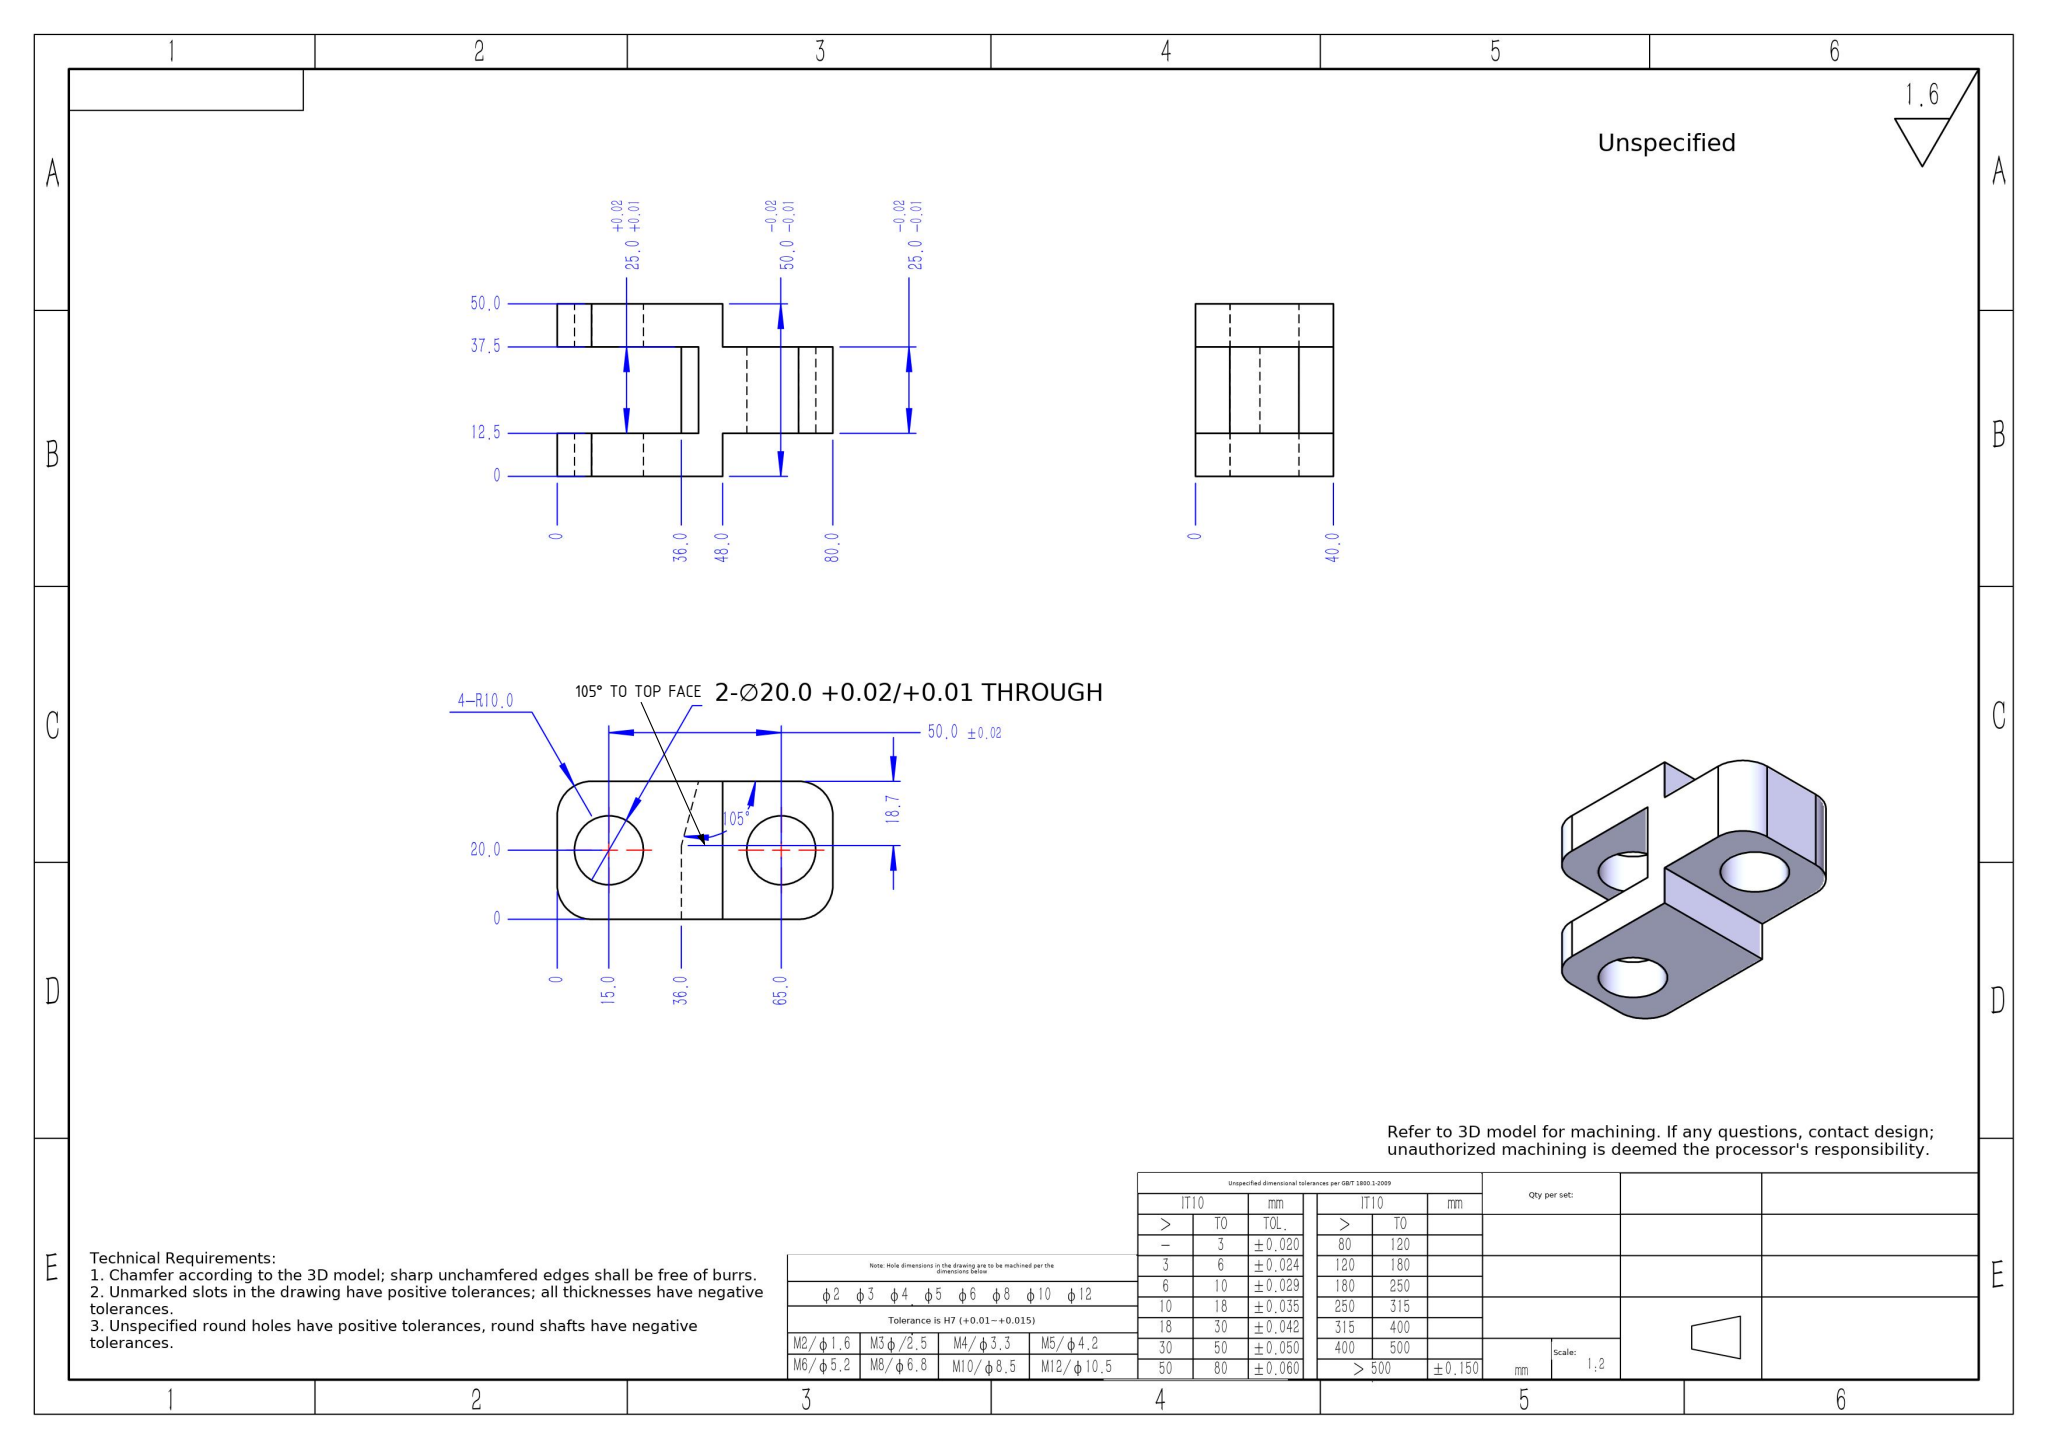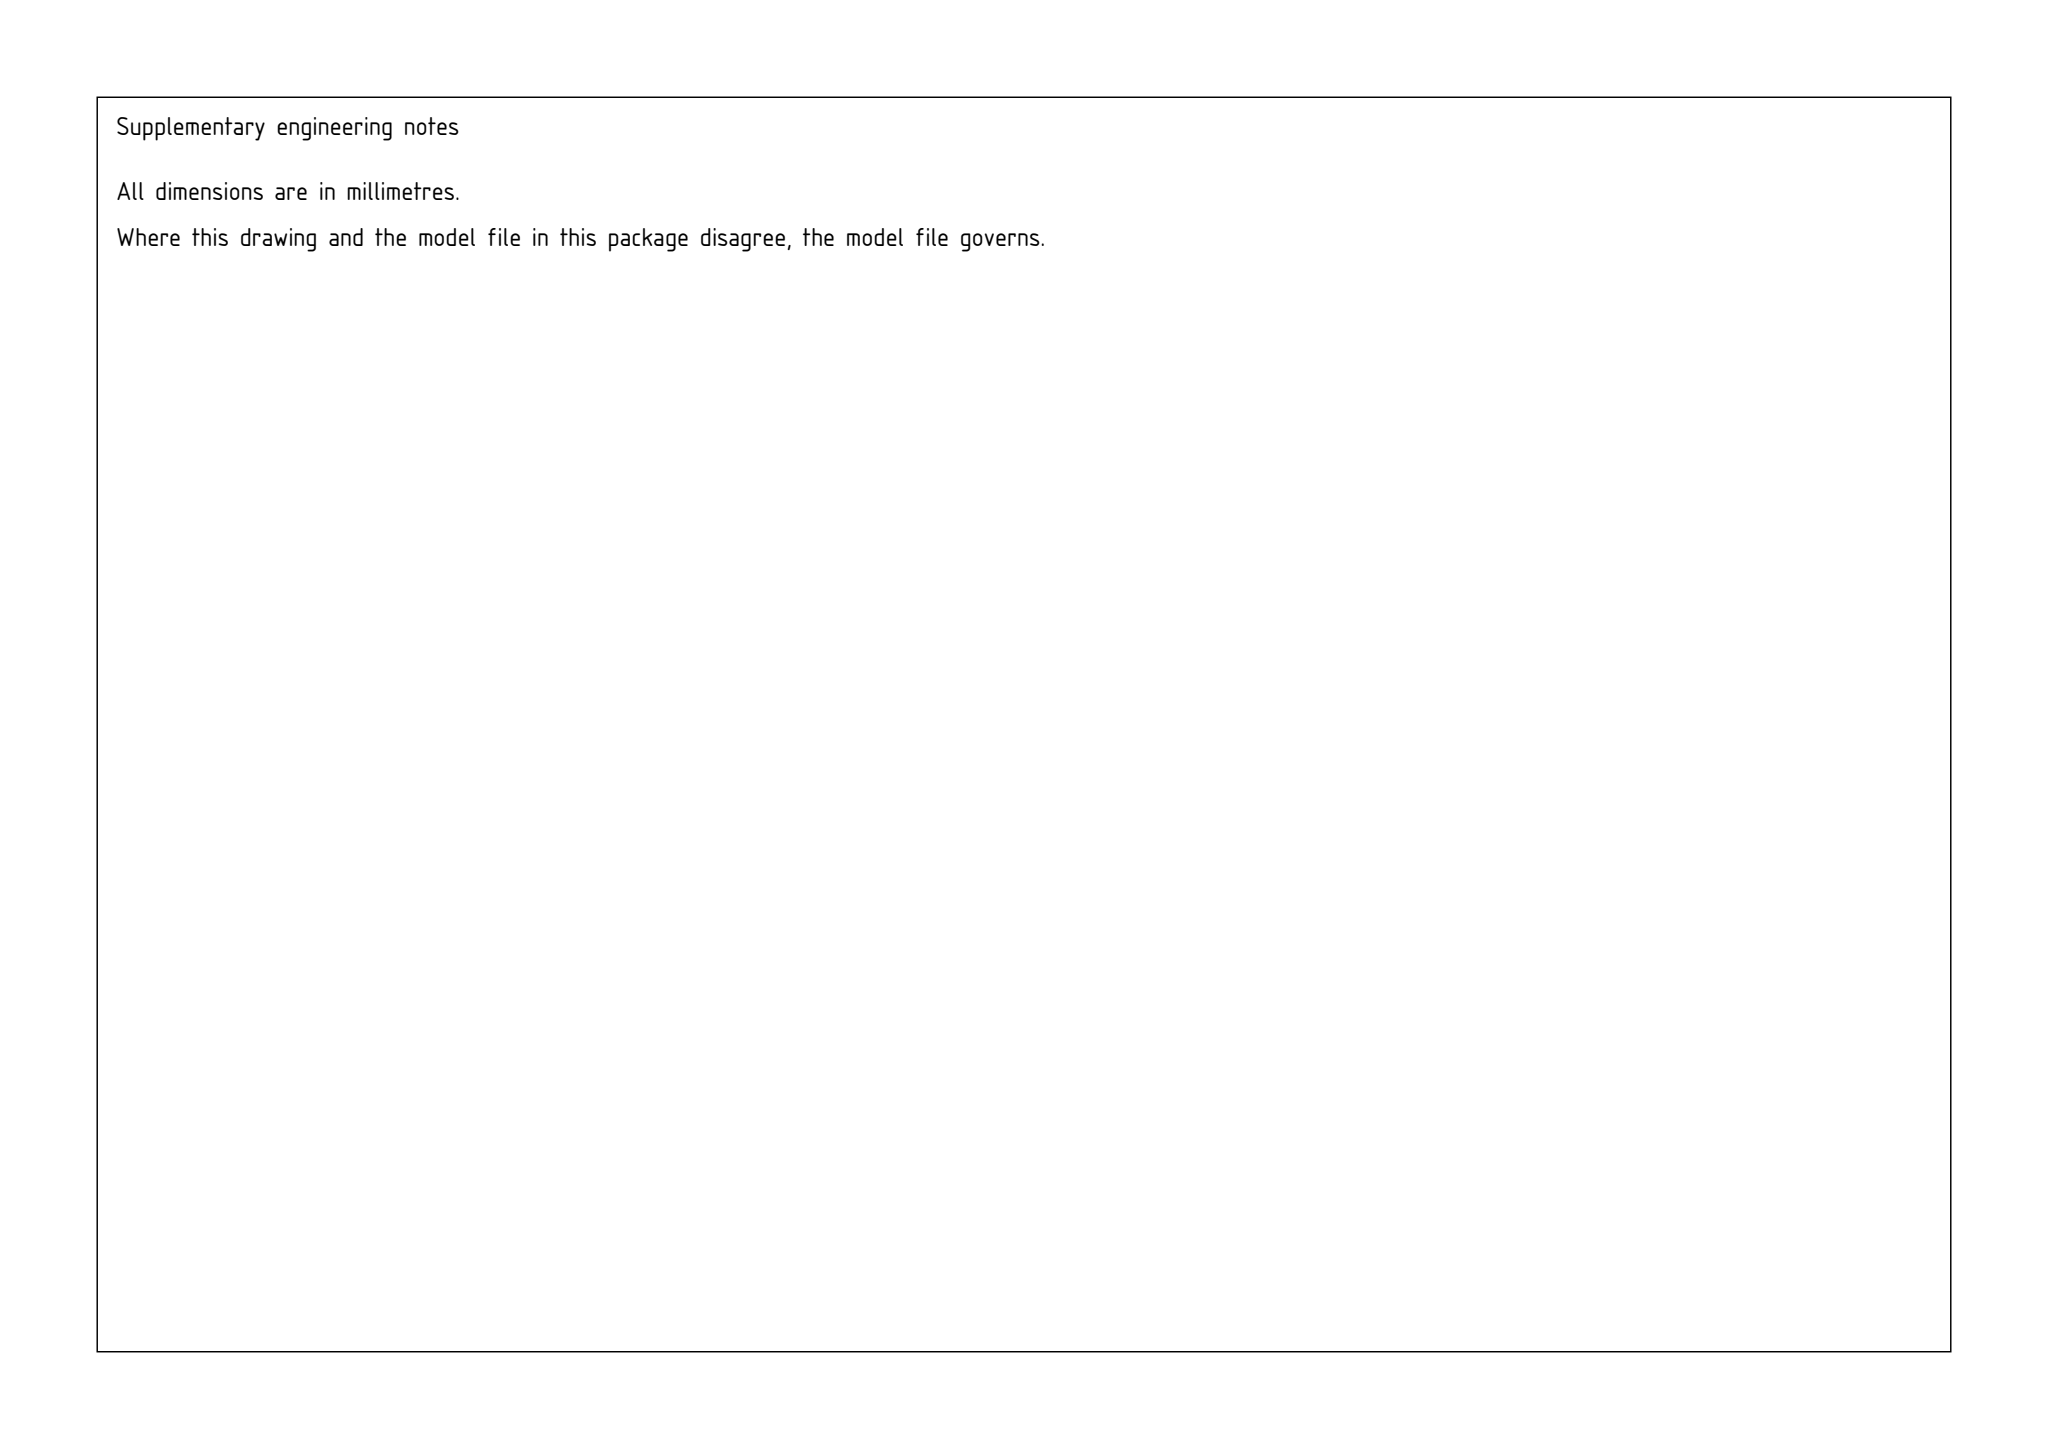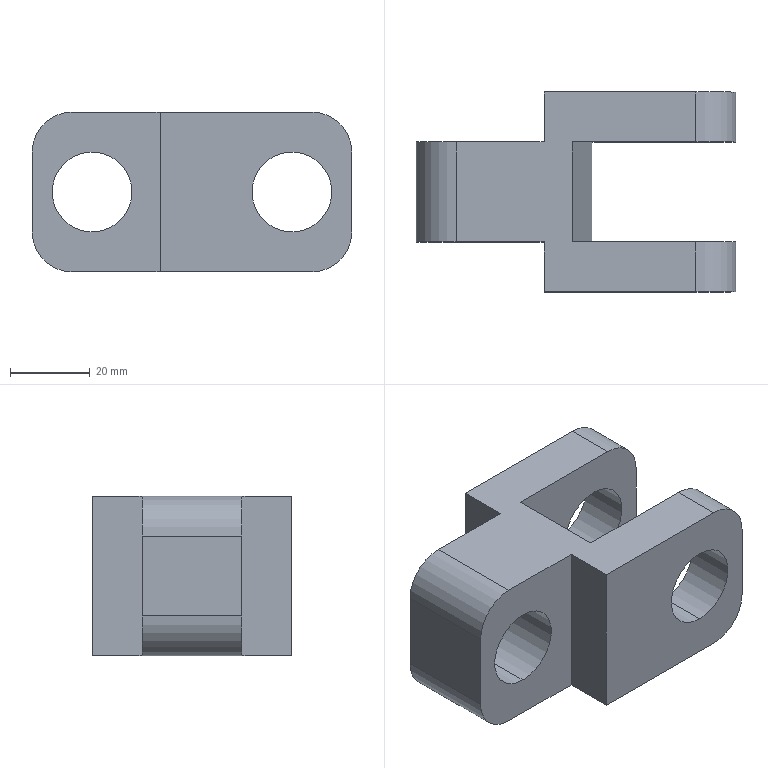Part | SolidWorks | mm | 1 solid | 27 faces | box 80 x 50 x 40 mm | volume 72980 mm3 | plane 15 | cylinder 12 | commonest cylinder face diameters 20 x12
Drawing notes:
ANGLED FACE 105° TO TOP FACE; RISE 18.7 OVER 5.0 RUN | from the solid: inclined plane angle_to_xyz [15,90,75], bbox_from [39,12.5,21.3], size [5,25,18.7]; 180-atan(18.7/5)=105° from top face z=40
build123d program:
from build123d import *

# Parameters (mm, degrees)
SKETCH1_W           = 80
SKETCH1_H           = 50
BOSS_EXTRUDE1_DEPTH = 20
SKETCH2_R           = 10
CUT_EXTRUDE1_DEPTH  = 205
SKETCH3_W           = 32
SKETCH3_H           = 40
CUT_EXTRUDE2_DEPTH  = 12.5
SKETCH4_W           = 36
SKETCH4_H           = 25
CUT_EXTRUDE3_DEPTH  = 256
FILLET1_R           = 10
CHAMFER1_SIZE       = 5
CHAMFER1_SIZE2      = 18.66


with BuildPart() as part:
    # Sketch1 → Boss-Extrude1 (new, symmetric)
    with BuildSketch(Plane.XY):
        Rectangle(SKETCH1_W, SKETCH1_H)
    extrude(amount=BOSS_EXTRUDE1_DEPTH, both=True)

    # Sketch2 → Cut-Extrude1 (cut)
    with BuildSketch(Plane.XZ.offset(25)):
        with Locations(Location((25, 0, 0), (0, 0, 270))):
            Circle(SKETCH2_R)
    cut_extrude1 = extrude(amount=-CUT_EXTRUDE1_DEPTH, mode=Mode.SUBTRACT)

    # Mirror1: Cut-Extrude1 across plane
    add(cut_extrude1.mirror(Plane(origin=(0, 0, 0), x_dir=(0, 0, 1), z_dir=(1, 0, 0))), mode=Mode.SUBTRACT)

    # Sketch3 → Cut-Extrude2 (cut)
    with BuildSketch(Plane.XZ.offset(25)):
        with Locations((-24, 0)):
            Rectangle(SKETCH3_W, SKETCH3_H)
    cut_extrude2 = extrude(amount=-CUT_EXTRUDE2_DEPTH, mode=Mode.SUBTRACT)

    # Mirror2: Cut-Extrude2 across plane
    add(cut_extrude2.mirror(Plane.ZX), mode=Mode.SUBTRACT)

    # Sketch4 → Cut-Extrude3 (cut)
    with BuildSketch(Plane(origin=(0, 0, -20), x_dir=(-1, 0, 0), z_dir=(0, 0, -1))):
        with Locations((-22, 0)):
            Rectangle(SKETCH4_W, SKETCH4_H)
    extrude(amount=-CUT_EXTRUDE3_DEPTH, mode=Mode.SUBTRACT)

    # Fillet1
    fillet1_edges = [part.edges().sort_by_distance(p)[0] for p in [
        (40, -18.75, 20),
        (-40, 0, -20),
        (-40, 0, 20),
        (40, -18.75, -20),
        (40, 18.75, -20),
        (40, 18.75, 20),
    ]]
    fillet(fillet1_edges, radius=FILLET1_R)

    # Chamfer1
    chamfer1_edges = [part.edges().sort_by_distance(p)[0] for p in [
        (4, 0, 20),
    ]]
    chamfer1_side = [part.faces().sort_by_distance(p)[0] for p in [
        (-0.3333, 0, 20),
    ]]
    chamfer(chamfer1_edges, length=CHAMFER1_SIZE, length2=CHAMFER1_SIZE2, reference=chamfer1_side[0])


solid = part.part
STEP:
#1=CARTESIAN_POINT('',(25.,-12.5,-10.));
#2=VERTEX_POINT('',#1);
#3=CARTESIAN_POINT('',(25.,-12.5,10.));
#4=VERTEX_POINT('',#3);
#5=CARTESIAN_POINT('',(25.,-12.5,0.));
#6=DIRECTION('',(0.,1.,0.));
#7=DIRECTION('',(0.,0.,-1.));
#8=AXIS2_PLACEMENT_3D('',#5,#6,#7);
#9=CIRCLE('',#8,10.);
#10=EDGE_CURVE('',#2,#4,#9,.T.);
#11=ORIENTED_EDGE('',*,*,#10,.T.);
#12=CARTESIAN_POINT('',(25.,-25.,10.));
#13=VERTEX_POINT('',#12);
#14=CARTESIAN_POINT('',(25.,180.,10.));
#15=DIRECTION('',(0.,-1.,0.));
#16=VECTOR('',#15,1000.);
#17=LINE('',#14,#16);
#18=EDGE_CURVE('',#4,#13,#17,.T.);
#19=ORIENTED_EDGE('',*,*,#18,.T.);
#20=CARTESIAN_POINT('',(25.,-25.,-10.));
#21=VERTEX_POINT('',#20);
#22=CARTESIAN_POINT('',(25.,-25.,0.));
#23=DIRECTION('',(0.,-1.,0.));
#24=DIRECTION('',(0.,0.,-1.));
#25=AXIS2_PLACEMENT_3D('',#22,#23,#24);
#26=CIRCLE('',#25,10.);
#27=EDGE_CURVE('',#13,#21,#26,.T.);
#28=ORIENTED_EDGE('',*,*,#27,.T.);
#29=CARTESIAN_POINT('',(25.,180.,-10.));
#30=DIRECTION('',(0.,-1.,0.));
#31=VECTOR('',#30,1000.);
#32=LINE('',#29,#31);
#33=EDGE_CURVE('',#2,#21,#32,.T.);
#34=ORIENTED_EDGE('',*,*,#33,.F.);
#35=EDGE_LOOP('',(#11,#19,#28,#34));
#36=FACE_OUTER_BOUND('',#35,.T.);
#37=CARTESIAN_POINT('',(25.,180.,0.));
#38=DIRECTION('',(0.,-1.,0.));
#39=DIRECTION('',(0.,0.,-1.));
#40=AXIS2_PLACEMENT_3D('',#37,#38,#39);
#41=CYLINDRICAL_SURFACE('',#40,10.);
#42=ADVANCED_FACE('',(#36),#41,.F.);
#43=CARTESIAN_POINT('',(-25.,12.5,-10.));
#44=VERTEX_POINT('',#43);
#45=CARTESIAN_POINT('',(-25.,12.5,10.));
#46=VERTEX_POINT('',#45);
#47=CARTESIAN_POINT('',(-25.,12.5,0.));
#48=DIRECTION('',(0.,1.,0.));
#49=DIRECTION('',(0.,0.,1.));
#50=AXIS2_PLACEMENT_3D('',#47,#48,#49);
#51=CIRCLE('',#50,10.);
#52=EDGE_CURVE('',#44,#46,#51,.T.);
#53=ORIENTED_EDGE('',*,*,#52,.T.);
#54=CARTESIAN_POINT('',(-25.,-12.5,10.));
#55=VERTEX_POINT('',#54);
#56=CARTESIAN_POINT('',(-25.,180.,10.));
#57=DIRECTION('',(0.,-1.,0.));
#58=VECTOR('',#57,1000.);
#59=LINE('',#56,#58);
#60=EDGE_CURVE('',#46,#55,#59,.T.);
#61=ORIENTED_EDGE('',*,*,#60,.T.);
#62=CARTESIAN_POINT('',(-25.,-12.5,-10.));
#63=VERTEX_POINT('',#62);
#64=CARTESIAN_POINT('',(-25.,-12.5,0.));
#65=DIRECTION('',(0.,-1.,0.));
#66=DIRECTION('',(0.,0.,-1.));
#67=AXIS2_PLACEMENT_3D('',#64,#65,#66);
#68=CIRCLE('',#67,10.);
#69=EDGE_CURVE('',#55,#63,#68,.T.);
#70=ORIENTED_EDGE('',*,*,#69,.T.);
#71=CARTESIAN_POINT('',(-25.,180.,-10.));
#72=DIRECTION('',(0.,-1.,0.));
#73=VECTOR('',#72,1000.);
#74=LINE('',#71,#73);
#75=EDGE_CURVE('',#44,#63,#74,.T.);
#76=ORIENTED_EDGE('',*,*,#75,.F.);
#77=EDGE_LOOP('',(#53,#61,#70,#76));
#78=FACE_OUTER_BOUND('',#77,.T.);
#79=CARTESIAN_POINT('',(-25.,180.,0.));
#80=DIRECTION('',(0.,-1.,0.));
#81=DIRECTION('',(0.,0.,-1.));
#82=AXIS2_PLACEMENT_3D('',#79,#80,#81);
#83=CYLINDRICAL_SURFACE('',#82,10.);
#84=ADVANCED_FACE('',(#78),#83,.F.);
#85=CARTESIAN_POINT('',(25.,25.,10.));
#86=VERTEX_POINT('',#85);
#87=CARTESIAN_POINT('',(25.,25.,-10.));
#88=VERTEX_POINT('',#87);
#89=CARTESIAN_POINT('',(25.,25.,0.));
#90=DIRECTION('',(0.,-1.,0.));
#91=DIRECTION('',(0.,0.,-1.));
#92=AXIS2_PLACEMENT_3D('',#89,#90,#91);
#93=CIRCLE('',#92,10.);
#94=EDGE_CURVE('',#86,#88,#93,.T.);
#95=ORIENTED_EDGE('',*,*,#94,.F.);
#96=CARTESIAN_POINT('',(25.,12.5,10.));
#97=VERTEX_POINT('',#96);
#98=CARTESIAN_POINT('',(25.,180.,10.));
#99=DIRECTION('',(0.,-1.,0.));
#100=VECTOR('',#99,1000.);
#101=LINE('',#98,#100);
#102=EDGE_CURVE('',#86,#97,#101,.T.);
#103=ORIENTED_EDGE('',*,*,#102,.T.);
#104=CARTESIAN_POINT('',(25.,12.5,-10.));
#105=VERTEX_POINT('',#104);
#106=CARTESIAN_POINT('',(25.,12.5,0.));
#107=DIRECTION('',(-0.,-1.,0.));
#108=DIRECTION('',(-1.,0.,0.));
#109=AXIS2_PLACEMENT_3D('',#106,#107,#108);
#110=CIRCLE('',#109,10.);
#111=EDGE_CURVE('',#97,#105,#110,.T.);
#112=ORIENTED_EDGE('',*,*,#111,.T.);
#113=CARTESIAN_POINT('',(25.,180.,-10.));
#114=DIRECTION('',(0.,-1.,0.));
#115=VECTOR('',#114,1000.);
#116=LINE('',#113,#115);
#117=EDGE_CURVE('',#88,#105,#116,.T.);
#118=ORIENTED_EDGE('',*,*,#117,.F.);
#119=EDGE_LOOP('',(#95,#103,#112,#118));
#120=FACE_OUTER_BOUND('',#119,.T.);
#121=CARTESIAN_POINT('',(25.,180.,0.));
#122=DIRECTION('',(0.,-1.,0.));
#123=DIRECTION('',(0.,0.,-1.));
#124=AXIS2_PLACEMENT_3D('',#121,#122,#123);
#125=CYLINDRICAL_SURFACE('',#124,10.);
#126=ADVANCED_FACE('',(#120),#125,.F.);
#127=CARTESIAN_POINT('',(40.,12.5,10.));
#128=VERTEX_POINT('',#127);
#129=CARTESIAN_POINT('',(40.,12.5,-10.));
#130=VERTEX_POINT('',#129);
#131=CARTESIAN_POINT('',(40.,12.5,236.));
#132=DIRECTION('',(0.,0.,-1.));
#133=VECTOR('',#132,1000.);
#134=LINE('',#131,#133);
#135=EDGE_CURVE('',#128,#130,#134,.T.);
#136=ORIENTED_EDGE('',*,*,#135,.T.);
#137=CARTESIAN_POINT('',(40.,25.,-10.));
#138=VERTEX_POINT('',#137);
#139=CARTESIAN_POINT('',(40.,25.,-10.));
#140=DIRECTION('',(0.,1.,0.));
#141=VECTOR('',#140,1000.);
#142=LINE('',#139,#141);
#143=EDGE_CURVE('',#130,#138,#142,.T.);
#144=ORIENTED_EDGE('',*,*,#143,.T.);
#145=CARTESIAN_POINT('',(40.,25.,10.));
#146=VERTEX_POINT('',#145);
#147=CARTESIAN_POINT('',(40.,25.,20.));
#148=DIRECTION('',(0.,0.,-1.));
#149=VECTOR('',#148,1000.);
#150=LINE('',#147,#149);
#151=EDGE_CURVE('',#146,#138,#150,.T.);
#152=ORIENTED_EDGE('',*,*,#151,.F.);
#153=CARTESIAN_POINT('',(40.,-25.,10.));
#154=DIRECTION('',(0.,-1.,0.));
#155=VECTOR('',#154,1000.);
#156=LINE('',#153,#155);
#157=EDGE_CURVE('',#146,#128,#156,.T.);
#158=ORIENTED_EDGE('',*,*,#157,.T.);
#159=EDGE_LOOP('',(#136,#144,#152,#158));
#160=FACE_OUTER_BOUND('',#159,.T.);
#161=CARTESIAN_POINT('',(40.,-25.,20.));
#162=DIRECTION('',(-1.,0.,0.));
#163=DIRECTION('',(0.,0.,1.));
#164=AXIS2_PLACEMENT_3D('',#161,#162,#163);
#165=PLANE('',#164);
#166=ADVANCED_FACE('',(#160),#165,.F.);
#167=ORIENTED_EDGE('',*,*,#102,.F.);
#168=CARTESIAN_POINT('',(25.,25.,0.));
#169=DIRECTION('',(0.,-1.,0.));
#170=DIRECTION('',(0.,0.,-1.));
#171=AXIS2_PLACEMENT_3D('',#168,#169,#170);
#172=CIRCLE('',#171,10.);
#173=EDGE_CURVE('',#88,#86,#172,.T.);
#174=ORIENTED_EDGE('',*,*,#173,.F.);
#175=ORIENTED_EDGE('',*,*,#117,.T.);
#176=CARTESIAN_POINT('',(25.,12.5,0.));
#177=DIRECTION('',(-0.,-1.,0.));
#178=DIRECTION('',(-1.,0.,0.));
#179=AXIS2_PLACEMENT_3D('',#176,#177,#178);
#180=CIRCLE('',#179,10.);
#181=EDGE_CURVE('',#105,#97,#180,.T.);
#182=ORIENTED_EDGE('',*,*,#181,.T.);
#183=EDGE_LOOP('',(#167,#174,#175,#182));
#184=FACE_OUTER_BOUND('',#183,.T.);
#185=CARTESIAN_POINT('',(25.,180.,0.));
#186=DIRECTION('',(0.,-1.,0.));
#187=DIRECTION('',(0.,0.,-1.));
#188=AXIS2_PLACEMENT_3D('',#185,#186,#187);
#189=CYLINDRICAL_SURFACE('',#188,10.);
#190=ADVANCED_FACE('',(#184),#189,.F.);
#191=CARTESIAN_POINT('',(-40.,12.5,10.));
#192=VERTEX_POINT('',#191);
#193=CARTESIAN_POINT('',(-40.,12.5,-10.));
#194=VERTEX_POINT('',#193);
#195=CARTESIAN_POINT('',(-40.,12.5,20.));
#196=DIRECTION('',(0.,0.,-1.));
#197=VECTOR('',#196,1000.);
#198=LINE('',#195,#197);
#199=EDGE_CURVE('',#192,#194,#198,.T.);
#200=ORIENTED_EDGE('',*,*,#199,.T.);
#201=CARTESIAN_POINT('',(-40.,-12.5,-10.));
#202=VERTEX_POINT('',#201);
#203=CARTESIAN_POINT('',(-40.,-12.5,-10.));
#204=DIRECTION('',(0.,-1.,0.));
#205=VECTOR('',#204,1000.);
#206=LINE('',#203,#205);
#207=EDGE_CURVE('',#194,#202,#206,.T.);
#208=ORIENTED_EDGE('',*,*,#207,.T.);
#209=CARTESIAN_POINT('',(-40.,-12.5,10.));
#210=VERTEX_POINT('',#209);
#211=CARTESIAN_POINT('',(-40.,-12.5,20.));
#212=DIRECTION('',(0.,0.,-1.));
#213=VECTOR('',#212,1000.);
#214=LINE('',#211,#213);
#215=EDGE_CURVE('',#210,#202,#214,.T.);
#216=ORIENTED_EDGE('',*,*,#215,.F.);
#217=CARTESIAN_POINT('',(-40.,-25.,10.));
#218=DIRECTION('',(0.,1.,0.));
#219=VECTOR('',#218,1000.);
#220=LINE('',#217,#219);
#221=EDGE_CURVE('',#210,#192,#220,.T.);
#222=ORIENTED_EDGE('',*,*,#221,.T.);
#223=EDGE_LOOP('',(#200,#208,#216,#222));
#224=FACE_OUTER_BOUND('',#223,.T.);
#225=CARTESIAN_POINT('',(-40.,-25.,20.));
#226=DIRECTION('',(1.,0.,0.));
#227=DIRECTION('',(0.,0.,-1.));
#228=AXIS2_PLACEMENT_3D('',#225,#226,#227);
#229=PLANE('',#228);
#230=ADVANCED_FACE('',(#224),#229,.F.);
#231=ORIENTED_EDGE('',*,*,#60,.F.);
#232=CARTESIAN_POINT('',(-25.,12.5,0.));
#233=DIRECTION('',(0.,1.,0.));
#234=DIRECTION('',(0.,0.,1.));
#235=AXIS2_PLACEMENT_3D('',#232,#233,#234);
#236=CIRCLE('',#235,10.);
#237=EDGE_CURVE('',#46,#44,#236,.T.);
#238=ORIENTED_EDGE('',*,*,#237,.T.);
#239=ORIENTED_EDGE('',*,*,#75,.T.);
#240=CARTESIAN_POINT('',(-25.,-12.5,0.));
#241=DIRECTION('',(0.,-1.,0.));
#242=DIRECTION('',(0.,0.,-1.));
#243=AXIS2_PLACEMENT_3D('',#240,#241,#242);
#244=CIRCLE('',#243,10.);
#245=EDGE_CURVE('',#63,#55,#244,.T.);
#246=ORIENTED_EDGE('',*,*,#245,.T.);
#247=EDGE_LOOP('',(#231,#238,#239,#246));
#248=FACE_OUTER_BOUND('',#247,.T.);
#249=CARTESIAN_POINT('',(-25.,180.,0.));
#250=DIRECTION('',(0.,-1.,0.));
#251=DIRECTION('',(0.,0.,-1.));
#252=AXIS2_PLACEMENT_3D('',#249,#250,#251);
#253=CYLINDRICAL_SURFACE('',#252,10.);
#254=ADVANCED_FACE('',(#248),#253,.F.);
#255=ORIENTED_EDGE('',*,*,#173,.T.);
#256=ORIENTED_EDGE('',*,*,#94,.T.);
#257=EDGE_LOOP('',(#255,#256));
#258=FACE_BOUND('',#257,.T.);
#259=ORIENTED_EDGE('',*,*,#151,.T.);
#260=CARTESIAN_POINT('',(30.,25.,-20.));
#261=VERTEX_POINT('',#260);
#262=CARTESIAN_POINT('',(30.,25.,-10.));
#263=DIRECTION('',(0.,1.,0.));
#264=DIRECTION('',(-0.,0.,-1.));
#265=AXIS2_PLACEMENT_3D('',#262,#263,#264);
#266=CIRCLE('',#265,10.);
#267=EDGE_CURVE('',#138,#261,#266,.T.);
#268=ORIENTED_EDGE('',*,*,#267,.T.);
#269=CARTESIAN_POINT('',(-8.,25.,-20.));
#270=VERTEX_POINT('',#269);
#271=CARTESIAN_POINT('',(-40.,25.,-20.));
#272=DIRECTION('',(-1.,0.,0.));
#273=VECTOR('',#272,1000.);
#274=LINE('',#271,#273);
#275=EDGE_CURVE('',#261,#270,#274,.T.);
#276=ORIENTED_EDGE('',*,*,#275,.T.);
#277=CARTESIAN_POINT('',(-8.,25.,20.));
#278=VERTEX_POINT('',#277);
#279=CARTESIAN_POINT('',(-8.,25.,20.));
#280=DIRECTION('',(-0.,0.,1.));
#281=VECTOR('',#280,1000.);
#282=LINE('',#279,#281);
#283=EDGE_CURVE('',#270,#278,#282,.T.);
#284=ORIENTED_EDGE('',*,*,#283,.T.);
#285=CARTESIAN_POINT('',(30.,25.,20.));
#286=VERTEX_POINT('',#285);
#287=CARTESIAN_POINT('',(-40.,25.,20.));
#288=DIRECTION('',(-1.,0.,0.));
#289=VECTOR('',#288,1000.);
#290=LINE('',#287,#289);
#291=EDGE_CURVE('',#286,#278,#290,.T.);
#292=ORIENTED_EDGE('',*,*,#291,.F.);
#293=CARTESIAN_POINT('',(30.,25.,10.));
#294=DIRECTION('',(0.,1.,0.));
#295=DIRECTION('',(0.,0.,-1.));
#296=AXIS2_PLACEMENT_3D('',#293,#294,#295);
#297=CIRCLE('',#296,10.);
#298=EDGE_CURVE('',#286,#146,#297,.T.);
#299=ORIENTED_EDGE('',*,*,#298,.T.);
#300=EDGE_LOOP('',(#259,#268,#276,#284,#292,#299));
#301=FACE_OUTER_BOUND('',#300,.T.);
#302=CARTESIAN_POINT('',(-40.,25.,20.));
#303=DIRECTION('',(0.,-1.,0.));
#304=DIRECTION('',(0.,0.,-1.));
#305=AXIS2_PLACEMENT_3D('',#302,#303,#304);
#306=PLANE('',#305);
#307=ADVANCED_FACE('',(#258,#301),#306,.F.);
#308=CARTESIAN_POINT('',(-1.,-12.5,20.));
#309=VERTEX_POINT('',#308);
#310=CARTESIAN_POINT('',(-1.,12.5,20.));
#311=VERTEX_POINT('',#310);
#312=CARTESIAN_POINT('',(-1.,0.,20.));
#313=DIRECTION('',(0.,1.,0.));
#314=VECTOR('',#313,1000.);
#315=LINE('',#312,#314);
#316=EDGE_CURVE('',#309,#311,#315,.T.);
#317=ORIENTED_EDGE('',*,*,#316,.T.);
#318=CARTESIAN_POINT('',(30.,12.5,20.));
#319=VERTEX_POINT('',#318);
#320=CARTESIAN_POINT('',(0.,12.5,20.));
#321=DIRECTION('',(1.,-0.,0.));
#322=VECTOR('',#321,1000.);
#323=LINE('',#320,#322);
#324=EDGE_CURVE('',#311,#319,#323,.T.);
#325=ORIENTED_EDGE('',*,*,#324,.T.);
#326=CARTESIAN_POINT('',(30.,0.,20.));
#327=DIRECTION('',(0.,1.,0.));
#328=VECTOR('',#327,1000.);
#329=LINE('',#326,#328);
#330=EDGE_CURVE('',#319,#286,#329,.T.);
#331=ORIENTED_EDGE('',*,*,#330,.T.);
#332=ORIENTED_EDGE('',*,*,#291,.T.);
#333=CARTESIAN_POINT('',(-8.,12.5,20.));
#334=VERTEX_POINT('',#333);
#335=CARTESIAN_POINT('',(-8.,12.5,20.));
#336=DIRECTION('',(0.,1.,0.));
#337=VECTOR('',#336,1000.);
#338=LINE('',#335,#337);
#339=EDGE_CURVE('',#334,#278,#338,.T.);
#340=ORIENTED_EDGE('',*,*,#339,.F.);
#341=CARTESIAN_POINT('',(-30.,12.5,20.));
#342=VERTEX_POINT('',#341);
#343=CARTESIAN_POINT('',(-40.,12.5,20.));
#344=DIRECTION('',(-1.,0.,0.));
#345=VECTOR('',#344,1000.);
#346=LINE('',#343,#345);
#347=EDGE_CURVE('',#334,#342,#346,.T.);
#348=ORIENTED_EDGE('',*,*,#347,.T.);
#349=CARTESIAN_POINT('',(-30.,-12.5,20.));
#350=VERTEX_POINT('',#349);
#351=CARTESIAN_POINT('',(-30.,0.,20.));
#352=DIRECTION('',(0.,-1.,0.));
#353=VECTOR('',#352,1000.);
#354=LINE('',#351,#353);
#355=EDGE_CURVE('',#342,#350,#354,.T.);
#356=ORIENTED_EDGE('',*,*,#355,.T.);
#357=CARTESIAN_POINT('',(-8.,-12.5,20.));
#358=VERTEX_POINT('',#357);
#359=CARTESIAN_POINT('',(-40.,-12.5,20.));
#360=DIRECTION('',(-1.,0.,0.));
#361=VECTOR('',#360,1000.);
#362=LINE('',#359,#361);
#363=EDGE_CURVE('',#358,#350,#362,.T.);
#364=ORIENTED_EDGE('',*,*,#363,.F.);
#365=CARTESIAN_POINT('',(-8.,-25.,20.));
#366=VERTEX_POINT('',#365);
#367=CARTESIAN_POINT('',(-8.,-12.5,20.));
#368=DIRECTION('',(0.,-1.,0.));
#369=VECTOR('',#368,1000.);
#370=LINE('',#367,#369);
#371=EDGE_CURVE('',#358,#366,#370,.T.);
#372=ORIENTED_EDGE('',*,*,#371,.T.);
#373=CARTESIAN_POINT('',(30.,-25.,20.));
#374=VERTEX_POINT('',#373);
#375=CARTESIAN_POINT('',(-40.,-25.,20.));
#376=DIRECTION('',(1.,0.,0.));
#377=VECTOR('',#376,1000.);
#378=LINE('',#375,#377);
#379=EDGE_CURVE('',#366,#374,#378,.T.);
#380=ORIENTED_EDGE('',*,*,#379,.T.);
#381=CARTESIAN_POINT('',(30.,-12.5,20.));
#382=VERTEX_POINT('',#381);
#383=CARTESIAN_POINT('',(30.,0.,20.));
#384=DIRECTION('',(0.,1.,0.));
#385=VECTOR('',#384,1000.);
#386=LINE('',#383,#385);
#387=EDGE_CURVE('',#374,#382,#386,.T.);
#388=ORIENTED_EDGE('',*,*,#387,.T.);
#389=CARTESIAN_POINT('',(0.,-12.5,20.));
#390=DIRECTION('',(-1.,0.,0.));
#391=VECTOR('',#390,1000.);
#392=LINE('',#389,#391);
#393=EDGE_CURVE('',#382,#309,#392,.T.);
#394=ORIENTED_EDGE('',*,*,#393,.T.);
#395=EDGE_LOOP('',(#317,#325,#331,#332,#340,#348,#356,#364,#372,#380,#388,#394));
#396=FACE_OUTER_BOUND('',#395,.T.);
#397=CARTESIAN_POINT('',(0.,0.,20.));
#398=DIRECTION('',(0.,0.,-1.));
#399=DIRECTION('',(-1.,0.,0.));
#400=AXIS2_PLACEMENT_3D('',#397,#398,#399);
#401=PLANE('',#400);
#402=ADVANCED_FACE('',(#396),#401,.F.);
#403=CARTESIAN_POINT('',(-30.,-12.5,-20.));
#404=VERTEX_POINT('',#403);
#405=CARTESIAN_POINT('',(-8.,-12.5,-20.));
#406=VERTEX_POINT('',#405);
#407=CARTESIAN_POINT('',(-40.,-12.5,-20.));
#408=DIRECTION('',(1.,0.,0.));
#409=VECTOR('',#408,1000.);
#410=LINE('',#407,#409);
#411=EDGE_CURVE('',#404,#406,#410,.T.);
#412=ORIENTED_EDGE('',*,*,#411,.F.);
#413=CARTESIAN_POINT('',(-30.,12.5,-20.));
#414=VERTEX_POINT('',#413);
#415=CARTESIAN_POINT('',(-30.,12.5,-20.));
#416=DIRECTION('',(0.,1.,0.));
#417=VECTOR('',#416,1000.);
#418=LINE('',#415,#417);
#419=EDGE_CURVE('',#404,#414,#418,.T.);
#420=ORIENTED_EDGE('',*,*,#419,.T.);
#421=CARTESIAN_POINT('',(-8.,12.5,-20.));
#422=VERTEX_POINT('',#421);
#423=CARTESIAN_POINT('',(-40.,12.5,-20.));
#424=DIRECTION('',(1.,0.,0.));
#425=VECTOR('',#424,1000.);
#426=LINE('',#423,#425);
#427=EDGE_CURVE('',#414,#422,#426,.T.);
#428=ORIENTED_EDGE('',*,*,#427,.T.);
#429=CARTESIAN_POINT('',(-8.,12.5,-20.));
#430=DIRECTION('',(0.,1.,0.));
#431=VECTOR('',#430,1000.);
#432=LINE('',#429,#431);
#433=EDGE_CURVE('',#422,#270,#432,.T.);
#434=ORIENTED_EDGE('',*,*,#433,.T.);
#435=ORIENTED_EDGE('',*,*,#275,.F.);
#436=CARTESIAN_POINT('',(30.,12.5,-20.));
#437=VERTEX_POINT('',#436);
#438=CARTESIAN_POINT('',(30.,12.5,-20.));
#439=DIRECTION('',(0.,-1.,0.));
#440=VECTOR('',#439,1000.);
#441=LINE('',#438,#440);
#442=EDGE_CURVE('',#261,#437,#441,.T.);
#443=ORIENTED_EDGE('',*,*,#442,.T.);
#444=CARTESIAN_POINT('',(4.,12.5,-20.));
#445=VERTEX_POINT('',#444);
#446=CARTESIAN_POINT('',(40.,12.5,-20.));
#447=DIRECTION('',(1.,-0.,0.));
#448=VECTOR('',#447,1000.);
#449=LINE('',#446,#448);
#450=EDGE_CURVE('',#445,#437,#449,.T.);
#451=ORIENTED_EDGE('',*,*,#450,.F.);
#452=CARTESIAN_POINT('',(4.,-12.5,-20.));
#453=VERTEX_POINT('',#452);
#454=CARTESIAN_POINT('',(4.,-12.5,-20.));
#455=DIRECTION('',(0.,1.,0.));
#456=VECTOR('',#455,1000.);
#457=LINE('',#454,#456);
#458=EDGE_CURVE('',#453,#445,#457,.T.);
#459=ORIENTED_EDGE('',*,*,#458,.F.);
#460=CARTESIAN_POINT('',(30.,-12.5,-20.));
#461=VERTEX_POINT('',#460);
#462=CARTESIAN_POINT('',(40.,-12.5,-20.));
#463=DIRECTION('',(-1.,0.,0.));
#464=VECTOR('',#463,1000.);
#465=LINE('',#462,#464);
#466=EDGE_CURVE('',#461,#453,#465,.T.);
#467=ORIENTED_EDGE('',*,*,#466,.F.);
#468=CARTESIAN_POINT('',(30.,-25.,-20.));
#469=VERTEX_POINT('',#468);
#470=CARTESIAN_POINT('',(30.,-25.,-20.));
#471=DIRECTION('',(0.,-1.,0.));
#472=VECTOR('',#471,1000.);
#473=LINE('',#470,#472);
#474=EDGE_CURVE('',#461,#469,#473,.T.);
#475=ORIENTED_EDGE('',*,*,#474,.T.);
#476=CARTESIAN_POINT('',(-8.,-25.,-20.));
#477=VERTEX_POINT('',#476);
#478=CARTESIAN_POINT('',(-40.,-25.,-20.));
#479=DIRECTION('',(1.,0.,0.));
#480=VECTOR('',#479,1000.);
#481=LINE('',#478,#480);
#482=EDGE_CURVE('',#477,#469,#481,.T.);
#483=ORIENTED_EDGE('',*,*,#482,.F.);
#484=CARTESIAN_POINT('',(-8.,-12.5,-20.));
#485=DIRECTION('',(0.,-1.,0.));
#486=VECTOR('',#485,1000.);
#487=LINE('',#484,#486);
#488=EDGE_CURVE('',#406,#477,#487,.T.);
#489=ORIENTED_EDGE('',*,*,#488,.F.);
#490=EDGE_LOOP('',(#412,#420,#428,#434,#435,#443,#451,#459,#467,#475,#483,#489));
#491=FACE_OUTER_BOUND('',#490,.T.);
#492=CARTESIAN_POINT('',(0.,0.,-20.));
#493=DIRECTION('',(0.,0.,-1.));
#494=DIRECTION('',(-1.,0.,0.));
#495=AXIS2_PLACEMENT_3D('',#492,#493,#494);
#496=PLANE('',#495);
#497=ADVANCED_FACE('',(#491),#496,.T.);
#498=CARTESIAN_POINT('',(40.,-25.,10.));
#499=VERTEX_POINT('',#498);
#500=CARTESIAN_POINT('',(40.,-25.,-10.));
#501=VERTEX_POINT('',#500);
#502=CARTESIAN_POINT('',(40.,-25.,20.));
#503=DIRECTION('',(0.,0.,-1.));
#504=VECTOR('',#503,1000.);
#505=LINE('',#502,#504);
#506=EDGE_CURVE('',#499,#501,#505,.T.);
#507=ORIENTED_EDGE('',*,*,#506,.T.);
#508=CARTESIAN_POINT('',(40.,-12.5,-10.));
#509=VERTEX_POINT('',#508);
#510=CARTESIAN_POINT('',(40.,-12.5,-10.));
#511=DIRECTION('',(0.,1.,0.));
#512=VECTOR('',#511,1000.);
#513=LINE('',#510,#512);
#514=EDGE_CURVE('',#501,#509,#513,.T.);
#515=ORIENTED_EDGE('',*,*,#514,.T.);
#516=CARTESIAN_POINT('',(40.,-12.5,10.));
#517=VERTEX_POINT('',#516);
#518=CARTESIAN_POINT('',(40.,-12.5,236.));
#519=DIRECTION('',(0.,0.,-1.));
#520=VECTOR('',#519,1000.);
#521=LINE('',#518,#520);
#522=EDGE_CURVE('',#517,#509,#521,.T.);
#523=ORIENTED_EDGE('',*,*,#522,.F.);
#524=CARTESIAN_POINT('',(40.,-25.,10.));
#525=DIRECTION('',(0.,-1.,0.));
#526=VECTOR('',#525,1000.);
#527=LINE('',#524,#526);
#528=EDGE_CURVE('',#517,#499,#527,.T.);
#529=ORIENTED_EDGE('',*,*,#528,.T.);
#530=EDGE_LOOP('',(#507,#515,#523,#529));
#531=FACE_OUTER_BOUND('',#530,.T.);
#532=CARTESIAN_POINT('',(40.,-25.,20.));
#533=DIRECTION('',(-1.,0.,0.));
#534=DIRECTION('',(0.,0.,1.));
#535=AXIS2_PLACEMENT_3D('',#532,#533,#534);
#536=PLANE('',#535);
#537=ADVANCED_FACE('',(#531),#536,.F.);
#538=CARTESIAN_POINT('',(25.,-25.,0.));
#539=DIRECTION('',(0.,-1.,0.));
#540=DIRECTION('',(0.,0.,-1.));
#541=AXIS2_PLACEMENT_3D('',#538,#539,#540);
#542=CIRCLE('',#541,10.);
#543=EDGE_CURVE('',#21,#13,#542,.T.);
#544=ORIENTED_EDGE('',*,*,#543,.F.);
#545=ORIENTED_EDGE('',*,*,#27,.F.);
#546=EDGE_LOOP('',(#544,#545));
#547=FACE_BOUND('',#546,.T.);
#548=ORIENTED_EDGE('',*,*,#482,.T.);
#549=CARTESIAN_POINT('',(30.,-25.,-10.));
#550=DIRECTION('',(0.,-1.,0.));
#551=DIRECTION('',(0.,0.,1.));
#552=AXIS2_PLACEMENT_3D('',#549,#550,#551);
#553=CIRCLE('',#552,10.);
#554=EDGE_CURVE('',#469,#501,#553,.T.);
#555=ORIENTED_EDGE('',*,*,#554,.T.);
#556=ORIENTED_EDGE('',*,*,#506,.F.);
#557=CARTESIAN_POINT('',(30.,-25.,10.));
#558=DIRECTION('',(0.,-1.,0.));
#559=DIRECTION('',(-0.,0.,1.));
#560=AXIS2_PLACEMENT_3D('',#557,#558,#559);
#561=CIRCLE('',#560,10.);
#562=EDGE_CURVE('',#499,#374,#561,.T.);
#563=ORIENTED_EDGE('',*,*,#562,.T.);
#564=ORIENTED_EDGE('',*,*,#379,.F.);
#565=CARTESIAN_POINT('',(-8.,-25.,20.));
#566=DIRECTION('',(-0.,0.,1.));
#567=VECTOR('',#566,1000.);
#568=LINE('',#565,#567);
#569=EDGE_CURVE('',#477,#366,#568,.T.);
#570=ORIENTED_EDGE('',*,*,#569,.F.);
#571=EDGE_LOOP('',(#548,#555,#556,#563,#564,#570));
#572=FACE_OUTER_BOUND('',#571,.T.);
#573=CARTESIAN_POINT('',(-40.,-25.,20.));
#574=DIRECTION('',(0.,1.,0.));
#575=DIRECTION('',(0.,0.,1.));
#576=AXIS2_PLACEMENT_3D('',#573,#574,#575);
#577=PLANE('',#576);
#578=ADVANCED_FACE('',(#547,#572),#577,.F.);
#579=ORIENTED_EDGE('',*,*,#18,.F.);
#580=CARTESIAN_POINT('',(25.,-12.5,0.));
#581=DIRECTION('',(0.,1.,0.));
#582=DIRECTION('',(0.,0.,-1.));
#583=AXIS2_PLACEMENT_3D('',#580,#581,#582);
#584=CIRCLE('',#583,10.);
#585=EDGE_CURVE('',#4,#2,#584,.T.);
#586=ORIENTED_EDGE('',*,*,#585,.T.);
#587=ORIENTED_EDGE('',*,*,#33,.T.);
#588=ORIENTED_EDGE('',*,*,#543,.T.);
#589=EDGE_LOOP('',(#579,#586,#587,#588));
#590=FACE_OUTER_BOUND('',#589,.T.);
#591=CARTESIAN_POINT('',(25.,180.,0.));
#592=DIRECTION('',(0.,-1.,0.));
#593=DIRECTION('',(0.,0.,-1.));
#594=AXIS2_PLACEMENT_3D('',#591,#592,#593);
#595=CYLINDRICAL_SURFACE('',#594,10.);
#596=ADVANCED_FACE('',(#590),#595,.F.);
#597=ORIENTED_EDGE('',*,*,#569,.T.);
#598=ORIENTED_EDGE('',*,*,#371,.F.);
#599=CARTESIAN_POINT('',(-8.,-12.5,20.));
#600=DIRECTION('',(-0.,0.,1.));
#601=VECTOR('',#600,1000.);
#602=LINE('',#599,#601);
#603=EDGE_CURVE('',#406,#358,#602,.T.);
#604=ORIENTED_EDGE('',*,*,#603,.F.);
#605=ORIENTED_EDGE('',*,*,#488,.T.);
#606=EDGE_LOOP('',(#597,#598,#604,#605));
#607=FACE_OUTER_BOUND('',#606,.T.);
#608=CARTESIAN_POINT('',(-8.,-12.5,20.));
#609=DIRECTION('',(1.,0.,0.));
#610=DIRECTION('',(0.,0.,-1.));
#611=AXIS2_PLACEMENT_3D('',#608,#609,#610);
#612=PLANE('',#611);
#613=ADVANCED_FACE('',(#607),#612,.F.);
#614=ORIENTED_EDGE('',*,*,#245,.F.);
#615=ORIENTED_EDGE('',*,*,#69,.F.);
#616=EDGE_LOOP('',(#614,#615));
#617=FACE_BOUND('',#616,.T.);
#618=ORIENTED_EDGE('',*,*,#215,.T.);
#619=CARTESIAN_POINT('',(-30.,-12.5,-10.));
#620=DIRECTION('',(0.,-1.,0.));
#621=DIRECTION('',(0.,0.,-1.));
#622=AXIS2_PLACEMENT_3D('',#619,#620,#621);
#623=CIRCLE('',#622,10.);
#624=EDGE_CURVE('',#202,#404,#623,.T.);
#625=ORIENTED_EDGE('',*,*,#624,.T.);
#626=ORIENTED_EDGE('',*,*,#411,.T.);
#627=ORIENTED_EDGE('',*,*,#603,.T.);
#628=ORIENTED_EDGE('',*,*,#363,.T.);
#629=CARTESIAN_POINT('',(-30.,-12.5,10.));
#630=DIRECTION('',(0.,-1.,0.));
#631=DIRECTION('',(0.,0.,-1.));
#632=AXIS2_PLACEMENT_3D('',#629,#630,#631);
#633=CIRCLE('',#632,10.);
#634=EDGE_CURVE('',#350,#210,#633,.T.);
#635=ORIENTED_EDGE('',*,*,#634,.T.);
#636=EDGE_LOOP('',(#618,#625,#626,#627,#628,#635));
#637=FACE_OUTER_BOUND('',#636,.T.);
#638=CARTESIAN_POINT('',(0.,-12.5,0.));
#639=DIRECTION('',(0.,-1.,0.));
#640=DIRECTION('',(0.,0.,-1.));
#641=AXIS2_PLACEMENT_3D('',#638,#639,#640);
#642=PLANE('',#641);
#643=ADVANCED_FACE('',(#617,#637),#642,.T.);
#644=ORIENTED_EDGE('',*,*,#283,.F.);
#645=ORIENTED_EDGE('',*,*,#433,.F.);
#646=CARTESIAN_POINT('',(-8.,12.5,20.));
#647=DIRECTION('',(-0.,0.,1.));
#648=VECTOR('',#647,1000.);
#649=LINE('',#646,#648);
#650=EDGE_CURVE('',#422,#334,#649,.T.);
#651=ORIENTED_EDGE('',*,*,#650,.T.);
#652=ORIENTED_EDGE('',*,*,#339,.T.);
#653=EDGE_LOOP('',(#644,#645,#651,#652));
#654=FACE_OUTER_BOUND('',#653,.T.);
#655=CARTESIAN_POINT('',(-8.,12.5,20.));
#656=DIRECTION('',(-1.,0.,-0.));
#657=DIRECTION('',(-0.,0.,1.));
#658=AXIS2_PLACEMENT_3D('',#655,#656,#657);
#659=PLANE('',#658);
#660=ADVANCED_FACE('',(#654),#659,.T.);
#661=ORIENTED_EDGE('',*,*,#52,.F.);
#662=ORIENTED_EDGE('',*,*,#237,.F.);
#663=EDGE_LOOP('',(#661,#662));
#664=FACE_BOUND('',#663,.T.);
#665=ORIENTED_EDGE('',*,*,#427,.F.);
#666=CARTESIAN_POINT('',(-30.,12.5,-10.));
#667=DIRECTION('',(0.,1.,0.));
#668=DIRECTION('',(0.,0.,1.));
#669=AXIS2_PLACEMENT_3D('',#666,#667,#668);
#670=CIRCLE('',#669,10.);
#671=EDGE_CURVE('',#414,#194,#670,.T.);
#672=ORIENTED_EDGE('',*,*,#671,.T.);
#673=ORIENTED_EDGE('',*,*,#199,.F.);
#674=CARTESIAN_POINT('',(-30.,12.5,10.));
#675=DIRECTION('',(0.,1.,0.));
#676=DIRECTION('',(0.,0.,1.));
#677=AXIS2_PLACEMENT_3D('',#674,#675,#676);
#678=CIRCLE('',#677,10.);
#679=EDGE_CURVE('',#192,#342,#678,.T.);
#680=ORIENTED_EDGE('',*,*,#679,.T.);
#681=ORIENTED_EDGE('',*,*,#347,.F.);
#682=ORIENTED_EDGE('',*,*,#650,.F.);
#683=EDGE_LOOP('',(#665,#672,#673,#680,#681,#682));
#684=FACE_OUTER_BOUND('',#683,.T.);
#685=CARTESIAN_POINT('',(0.,12.5,0.));
#686=DIRECTION('',(0.,1.,0.));
#687=DIRECTION('',(0.,0.,-1.));
#688=AXIS2_PLACEMENT_3D('',#685,#686,#687);
#689=PLANE('',#688);
#690=ADVANCED_FACE('',(#664,#684),#689,.T.);
#691=CARTESIAN_POINT('',(4.,12.5,1.34));
#692=VERTEX_POINT('',#691);
#693=CARTESIAN_POINT('',(4.,12.5,236.));
#694=DIRECTION('',(0.,0.,-1.));
#695=VECTOR('',#694,1000.);
#696=LINE('',#693,#695);
#697=EDGE_CURVE('',#692,#445,#696,.T.);
#698=ORIENTED_EDGE('',*,*,#697,.F.);
#699=CARTESIAN_POINT('',(4.,-12.5,1.34));
#700=VERTEX_POINT('',#699);
#701=CARTESIAN_POINT('',(4.,-12.5,1.34));
#702=DIRECTION('',(-0.,-1.,0.));
#703=VECTOR('',#702,1000.);
#704=LINE('',#701,#703);
#705=EDGE_CURVE('',#692,#700,#704,.T.);
#706=ORIENTED_EDGE('',*,*,#705,.T.);
#707=CARTESIAN_POINT('',(4.,-12.5,236.));
#708=DIRECTION('',(0.,0.,-1.));
#709=VECTOR('',#708,1000.);
#710=LINE('',#707,#709);
#711=EDGE_CURVE('',#700,#453,#710,.T.);
#712=ORIENTED_EDGE('',*,*,#711,.T.);
#713=ORIENTED_EDGE('',*,*,#458,.T.);
#714=EDGE_LOOP('',(#698,#706,#712,#713));
#715=FACE_OUTER_BOUND('',#714,.T.);
#716=CARTESIAN_POINT('',(4.,-12.5,236.));
#717=DIRECTION('',(-1.,0.,0.));
#718=DIRECTION('',(-0.,-1.,0.));
#719=AXIS2_PLACEMENT_3D('',#716,#717,#718);
#720=PLANE('',#719);
#721=ADVANCED_FACE('',(#715),#720,.F.);
#722=ORIENTED_EDGE('',*,*,#181,.F.);
#723=ORIENTED_EDGE('',*,*,#111,.F.);
#724=EDGE_LOOP('',(#722,#723));
#725=FACE_BOUND('',#724,.T.);
#726=ORIENTED_EDGE('',*,*,#450,.T.);
#727=CARTESIAN_POINT('',(30.,12.5,-10.));
#728=DIRECTION('',(-0.,-1.,0.));
#729=DIRECTION('',(-1.,0.,0.));
#730=AXIS2_PLACEMENT_3D('',#727,#728,#729);
#731=CIRCLE('',#730,10.);
#732=EDGE_CURVE('',#437,#130,#731,.T.);
#733=ORIENTED_EDGE('',*,*,#732,.T.);
#734=ORIENTED_EDGE('',*,*,#135,.F.);
#735=CARTESIAN_POINT('',(30.,12.5,10.));
#736=DIRECTION('',(-0.,-1.,0.));
#737=DIRECTION('',(-1.,0.,0.));
#738=AXIS2_PLACEMENT_3D('',#735,#736,#737);
#739=CIRCLE('',#738,10.);
#740=EDGE_CURVE('',#128,#319,#739,.T.);
#741=ORIENTED_EDGE('',*,*,#740,.T.);
#742=ORIENTED_EDGE('',*,*,#324,.F.);
#743=CARTESIAN_POINT('',(-52.254,12.5,211.281));
#744=DIRECTION('',(0.2588,-0.,-0.9659));
#745=VECTOR('',#744,1000.);
#746=LINE('',#743,#745);
#747=EDGE_CURVE('',#311,#692,#746,.T.);
#748=ORIENTED_EDGE('',*,*,#747,.T.);
#749=ORIENTED_EDGE('',*,*,#697,.T.);
#750=EDGE_LOOP('',(#726,#733,#734,#741,#742,#748,#749));
#751=FACE_OUTER_BOUND('',#750,.T.);
#752=CARTESIAN_POINT('',(40.,12.5,236.));
#753=DIRECTION('',(0.,1.,0.));
#754=DIRECTION('',(-1.,0.,0.));
#755=AXIS2_PLACEMENT_3D('',#752,#753,#754);
#756=PLANE('',#755);
#757=ADVANCED_FACE('',(#725,#751),#756,.F.);
#758=ORIENTED_EDGE('',*,*,#10,.F.);
#759=ORIENTED_EDGE('',*,*,#585,.F.);
#760=EDGE_LOOP('',(#758,#759));
#761=FACE_BOUND('',#760,.T.);
#762=ORIENTED_EDGE('',*,*,#522,.T.);
#763=CARTESIAN_POINT('',(30.,-12.5,-10.));
#764=DIRECTION('',(0.,1.,0.));
#765=DIRECTION('',(0.,0.,-1.));
#766=AXIS2_PLACEMENT_3D('',#763,#764,#765);
#767=CIRCLE('',#766,10.);
#768=EDGE_CURVE('',#509,#461,#767,.T.);
#769=ORIENTED_EDGE('',*,*,#768,.T.);
#770=ORIENTED_EDGE('',*,*,#466,.T.);
#771=ORIENTED_EDGE('',*,*,#711,.F.);
#772=CARTESIAN_POINT('',(-52.254,-12.5,211.281));
#773=DIRECTION('',(-0.2588,0.,0.9659));
#774=VECTOR('',#773,1000.);
#775=LINE('',#772,#774);
#776=EDGE_CURVE('',#700,#309,#775,.T.);
#777=ORIENTED_EDGE('',*,*,#776,.T.);
#778=ORIENTED_EDGE('',*,*,#393,.F.);
#779=CARTESIAN_POINT('',(30.,-12.5,10.));
#780=DIRECTION('',(0.,1.,0.));
#781=DIRECTION('',(0.,0.,-1.));
#782=AXIS2_PLACEMENT_3D('',#779,#780,#781);
#783=CIRCLE('',#782,10.);
#784=EDGE_CURVE('',#382,#517,#783,.T.);
#785=ORIENTED_EDGE('',*,*,#784,.T.);
#786=EDGE_LOOP('',(#762,#769,#770,#771,#777,#778,#785));
#787=FACE_OUTER_BOUND('',#786,.T.);
#788=CARTESIAN_POINT('',(40.,-12.5,236.));
#789=DIRECTION('',(0.,-1.,0.));
#790=DIRECTION('',(0.,0.,-1.));
#791=AXIS2_PLACEMENT_3D('',#788,#789,#790);
#792=PLANE('',#791);
#793=ADVANCED_FACE('',(#761,#787),#792,.F.);
#794=ORIENTED_EDGE('',*,*,#671,.F.);
#795=ORIENTED_EDGE('',*,*,#419,.F.);
#796=ORIENTED_EDGE('',*,*,#624,.F.);
#797=ORIENTED_EDGE('',*,*,#207,.F.);
#798=EDGE_LOOP('',(#794,#795,#796,#797));
#799=FACE_OUTER_BOUND('',#798,.T.);
#800=CARTESIAN_POINT('',(-30.,-25.,-10.));
#801=DIRECTION('',(0.,1.,0.));
#802=DIRECTION('',(0.,0.,1.));
#803=AXIS2_PLACEMENT_3D('',#800,#801,#802);
#804=CYLINDRICAL_SURFACE('',#803,10.);
#805=ADVANCED_FACE('',(#799),#804,.T.);
#806=ORIENTED_EDGE('',*,*,#679,.F.);
#807=ORIENTED_EDGE('',*,*,#221,.F.);
#808=ORIENTED_EDGE('',*,*,#634,.F.);
#809=ORIENTED_EDGE('',*,*,#355,.F.);
#810=EDGE_LOOP('',(#806,#807,#808,#809));
#811=FACE_OUTER_BOUND('',#810,.T.);
#812=CARTESIAN_POINT('',(-30.,0.,10.));
#813=DIRECTION('',(0.,-1.,0.));
#814=DIRECTION('',(0.,0.,-1.));
#815=AXIS2_PLACEMENT_3D('',#812,#813,#814);
#816=CYLINDRICAL_SURFACE('',#815,10.);
#817=ADVANCED_FACE('',(#811),#816,.T.);
#818=ORIENTED_EDGE('',*,*,#554,.F.);
#819=ORIENTED_EDGE('',*,*,#474,.F.);
#820=ORIENTED_EDGE('',*,*,#768,.F.);
#821=ORIENTED_EDGE('',*,*,#514,.F.);
#822=EDGE_LOOP('',(#818,#819,#820,#821));
#823=FACE_OUTER_BOUND('',#822,.T.);
#824=CARTESIAN_POINT('',(30.,-25.,-10.));
#825=DIRECTION('',(0.,-1.,0.));
#826=DIRECTION('',(0.,0.,-1.));
#827=AXIS2_PLACEMENT_3D('',#824,#825,#826);
#828=CYLINDRICAL_SURFACE('',#827,10.);
#829=ADVANCED_FACE('',(#823),#828,.T.);
#830=ORIENTED_EDGE('',*,*,#732,.F.);
#831=ORIENTED_EDGE('',*,*,#442,.F.);
#832=ORIENTED_EDGE('',*,*,#267,.F.);
#833=ORIENTED_EDGE('',*,*,#143,.F.);
#834=EDGE_LOOP('',(#830,#831,#832,#833));
#835=FACE_OUTER_BOUND('',#834,.T.);
#836=CARTESIAN_POINT('',(30.,-25.,-10.));
#837=DIRECTION('',(0.,-1.,0.));
#838=DIRECTION('',(0.,0.,-1.));
#839=AXIS2_PLACEMENT_3D('',#836,#837,#838);
#840=CYLINDRICAL_SURFACE('',#839,10.);
#841=ADVANCED_FACE('',(#835),#840,.T.);
#842=ORIENTED_EDGE('',*,*,#562,.F.);
#843=ORIENTED_EDGE('',*,*,#528,.F.);
#844=ORIENTED_EDGE('',*,*,#784,.F.);
#845=ORIENTED_EDGE('',*,*,#387,.F.);
#846=EDGE_LOOP('',(#842,#843,#844,#845));
#847=FACE_OUTER_BOUND('',#846,.T.);
#848=CARTESIAN_POINT('',(30.,0.,10.));
#849=DIRECTION('',(0.,1.,0.));
#850=DIRECTION('',(0.,0.,1.));
#851=AXIS2_PLACEMENT_3D('',#848,#849,#850);
#852=CYLINDRICAL_SURFACE('',#851,10.);
#853=ADVANCED_FACE('',(#847),#852,.T.);
#854=ORIENTED_EDGE('',*,*,#740,.F.);
#855=ORIENTED_EDGE('',*,*,#157,.F.);
#856=ORIENTED_EDGE('',*,*,#298,.F.);
#857=ORIENTED_EDGE('',*,*,#330,.F.);
#858=EDGE_LOOP('',(#854,#855,#856,#857));
#859=FACE_OUTER_BOUND('',#858,.T.);
#860=CARTESIAN_POINT('',(30.,0.,10.));
#861=DIRECTION('',(0.,1.,0.));
#862=DIRECTION('',(0.,0.,1.));
#863=AXIS2_PLACEMENT_3D('',#860,#861,#862);
#864=CYLINDRICAL_SURFACE('',#863,10.);
#865=ADVANCED_FACE('',(#859),#864,.T.);
#866=ORIENTED_EDGE('',*,*,#776,.F.);
#867=ORIENTED_EDGE('',*,*,#705,.F.);
#868=ORIENTED_EDGE('',*,*,#747,.F.);
#869=ORIENTED_EDGE('',*,*,#316,.F.);
#870=EDGE_LOOP('',(#866,#867,#868,#869));
#871=FACE_OUTER_BOUND('',#870,.T.);
#872=CARTESIAN_POINT('',(-1.,0.,20.));
#873=DIRECTION('',(-0.9659,0.,-0.2588));
#874=DIRECTION('',(0.,1.,0.));
#875=AXIS2_PLACEMENT_3D('',#872,#873,#874);
#876=PLANE('',#875);
#877=ADVANCED_FACE('',(#871),#876,.F.);
#878=CLOSED_SHELL('',(#42,#84,#126,#166,#190,#230,#254,#307,#402,#497,#537,#578,#596,#613,#643,#660,#690,#721,#757,#793,#805,#817,#829,#841,#853,#865,#877));
#879=MANIFOLD_SOLID_BREP('',#878);
#880=CARTESIAN_POINT('',(0.,0.,0.));
#881=DIRECTION('',(0.,0.,1.));
#882=DIRECTION('',(1.,0.,0.));
#883=AXIS2_PLACEMENT_3D('',#880,#881,#882);
#884=(LENGTH_UNIT()NAMED_UNIT(*)SI_UNIT(.MILLI.,.METRE.));
#885=UNCERTAINTY_MEASURE_WITH_UNIT(LENGTH_MEASURE(0.00001),#884,'','');
#886=(NAMED_UNIT(*)PLANE_ANGLE_UNIT()SI_UNIT($,.RADIAN.));
#887=(NAMED_UNIT(*)SI_UNIT($,.STERADIAN.)SOLID_ANGLE_UNIT());
#888=(GEOMETRIC_REPRESENTATION_CONTEXT(3)GLOBAL_UNCERTAINTY_ASSIGNED_CONTEXT((#885))GLOBAL_UNIT_ASSIGNED_CONTEXT((#884,#886,#887))REPRESENTATION_CONTEXT('',''));
#889=ADVANCED_BREP_SHAPE_REPRESENTATION('',(#879,#883),#888);